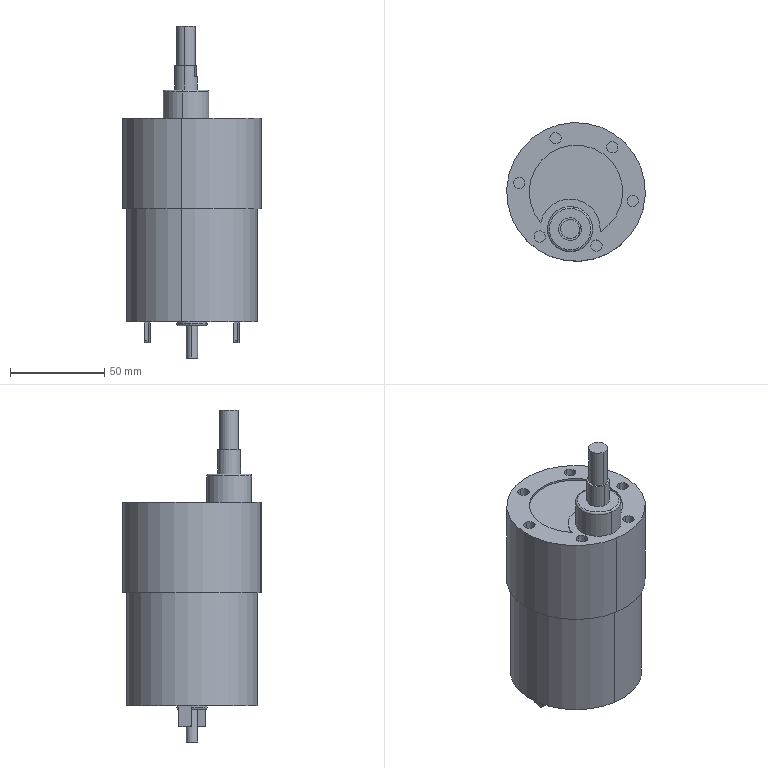Component | SolidWorks | DriveDevice-1_BrushedDCMotor-1 | 1 solid | 65 faces | volume 441088 mm3 | cylinder 34 | plane 27 | torus 4 | commonest cylinder face diameters 6 x14 2 x6 10 x2 16 x2 24 x2 69.6 x2 73.6 x2 12 x2